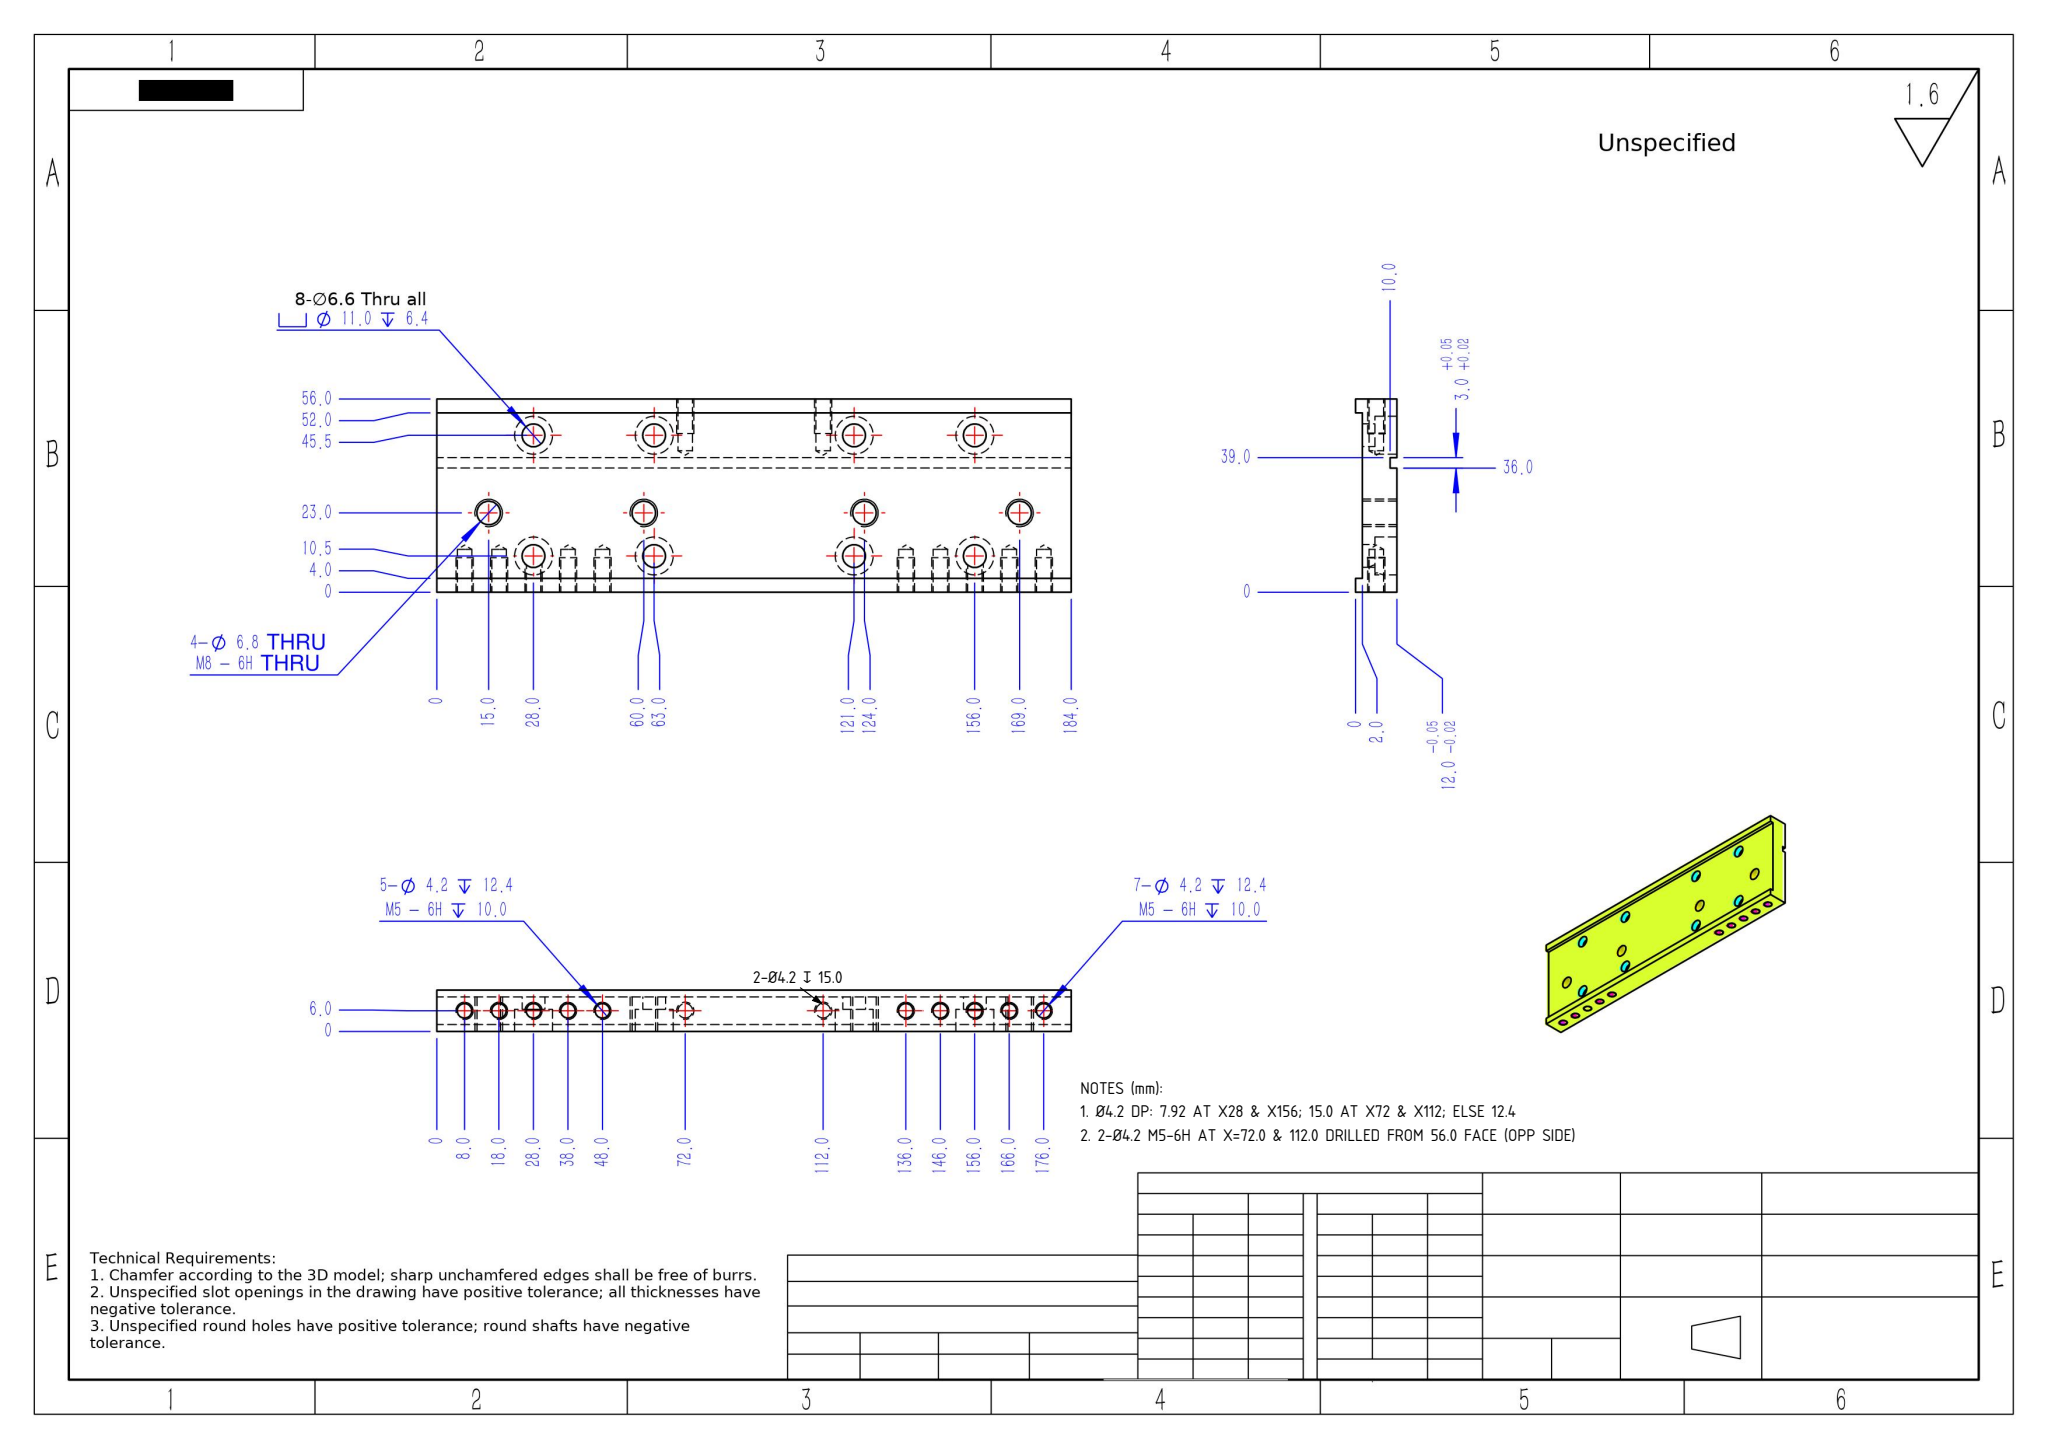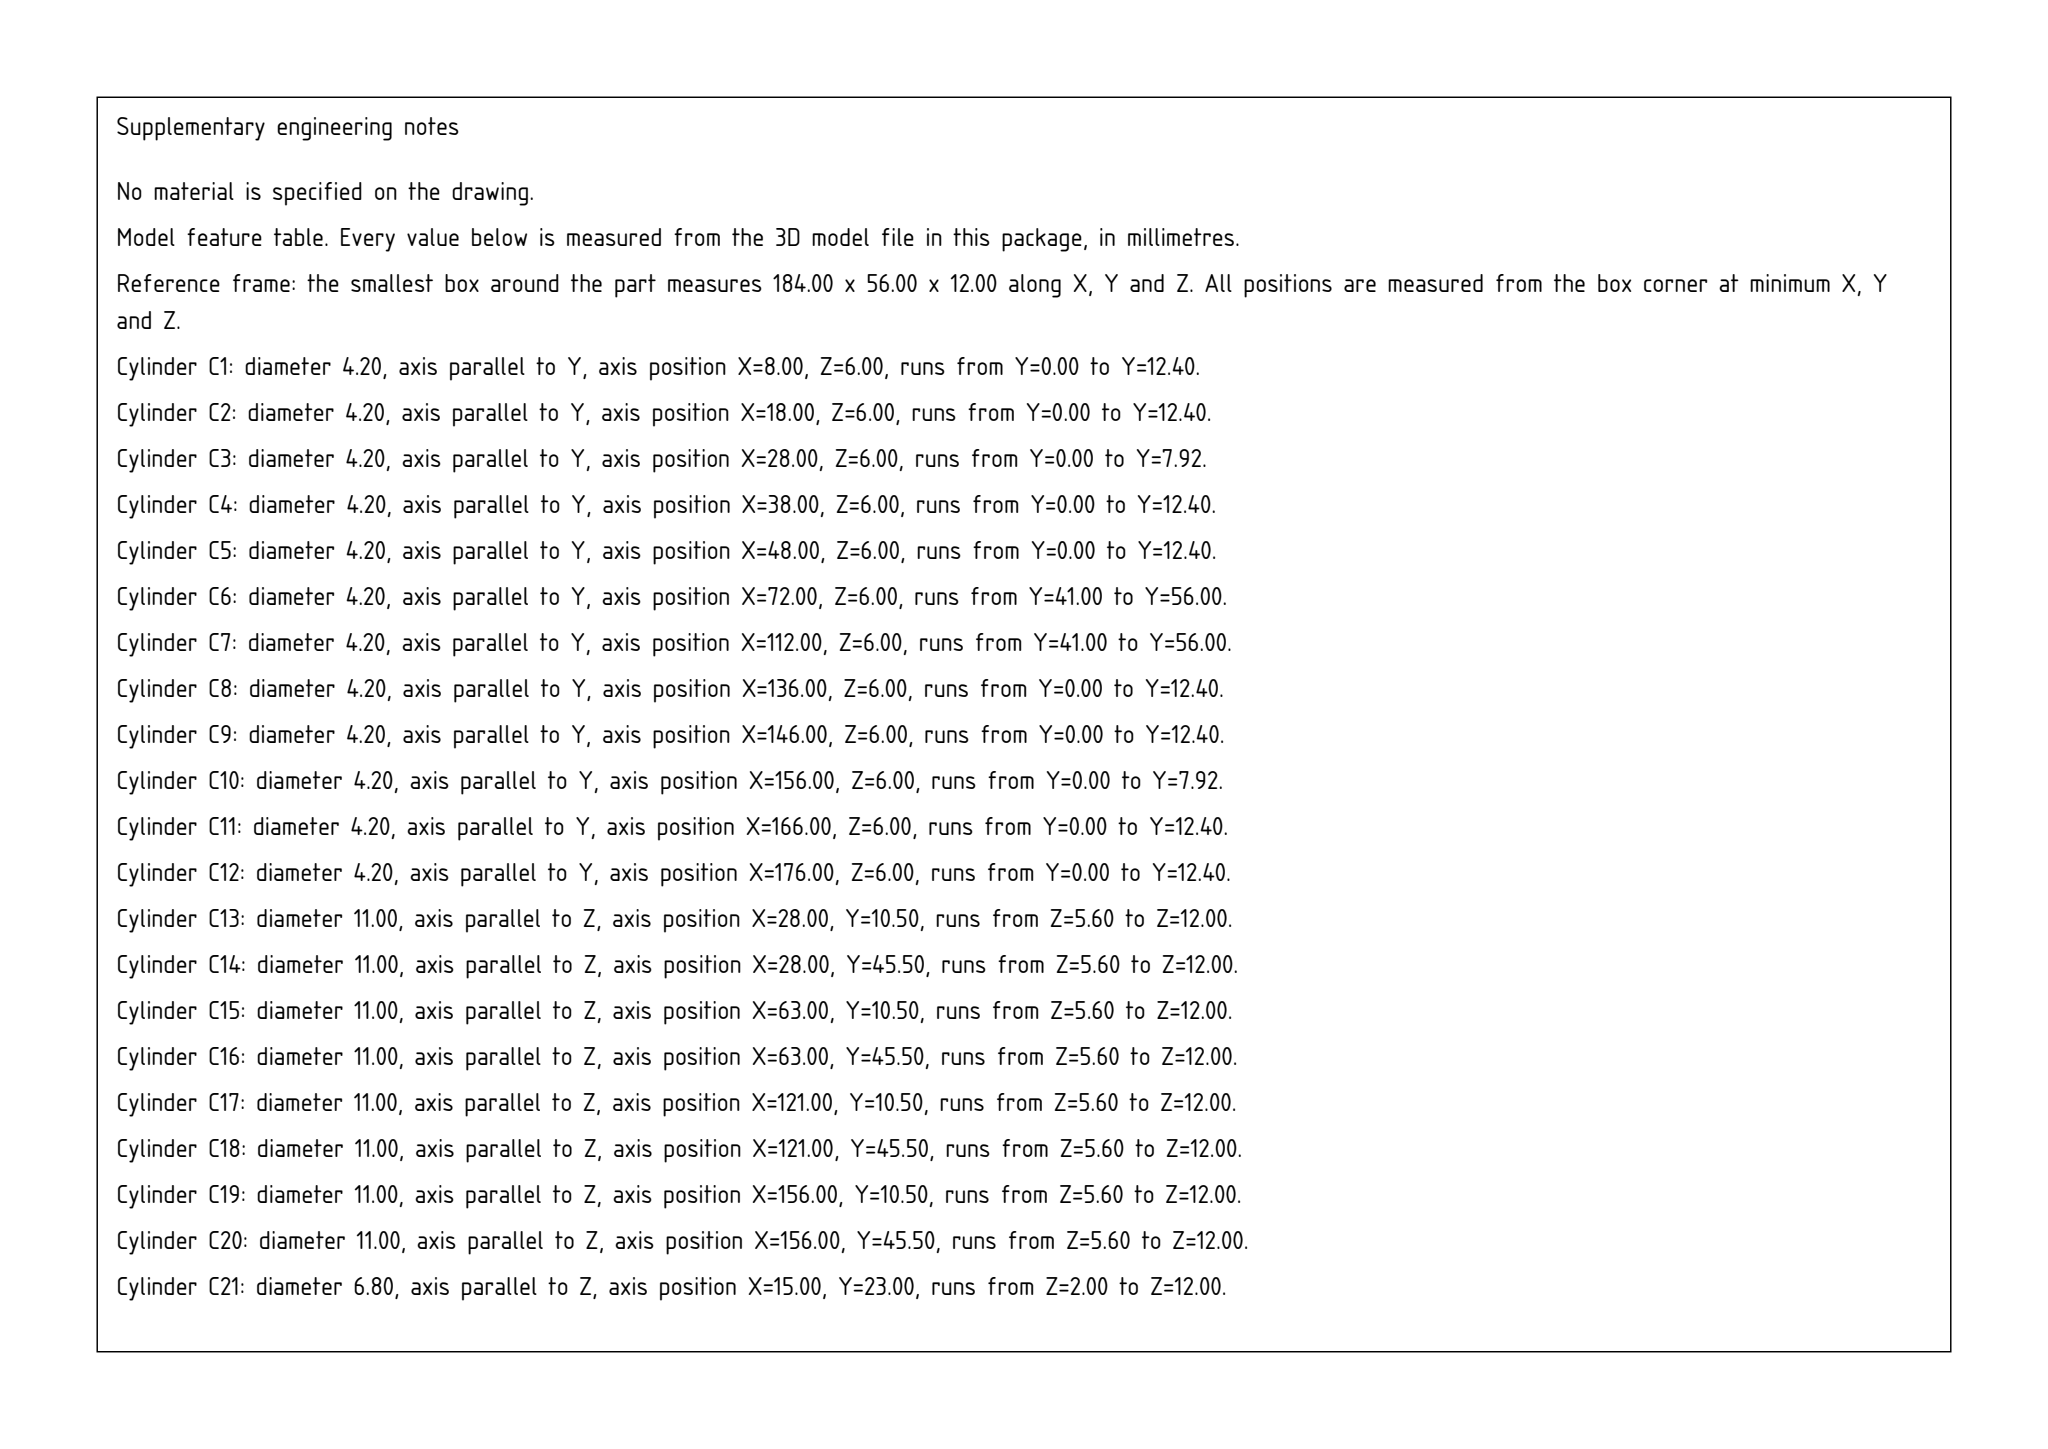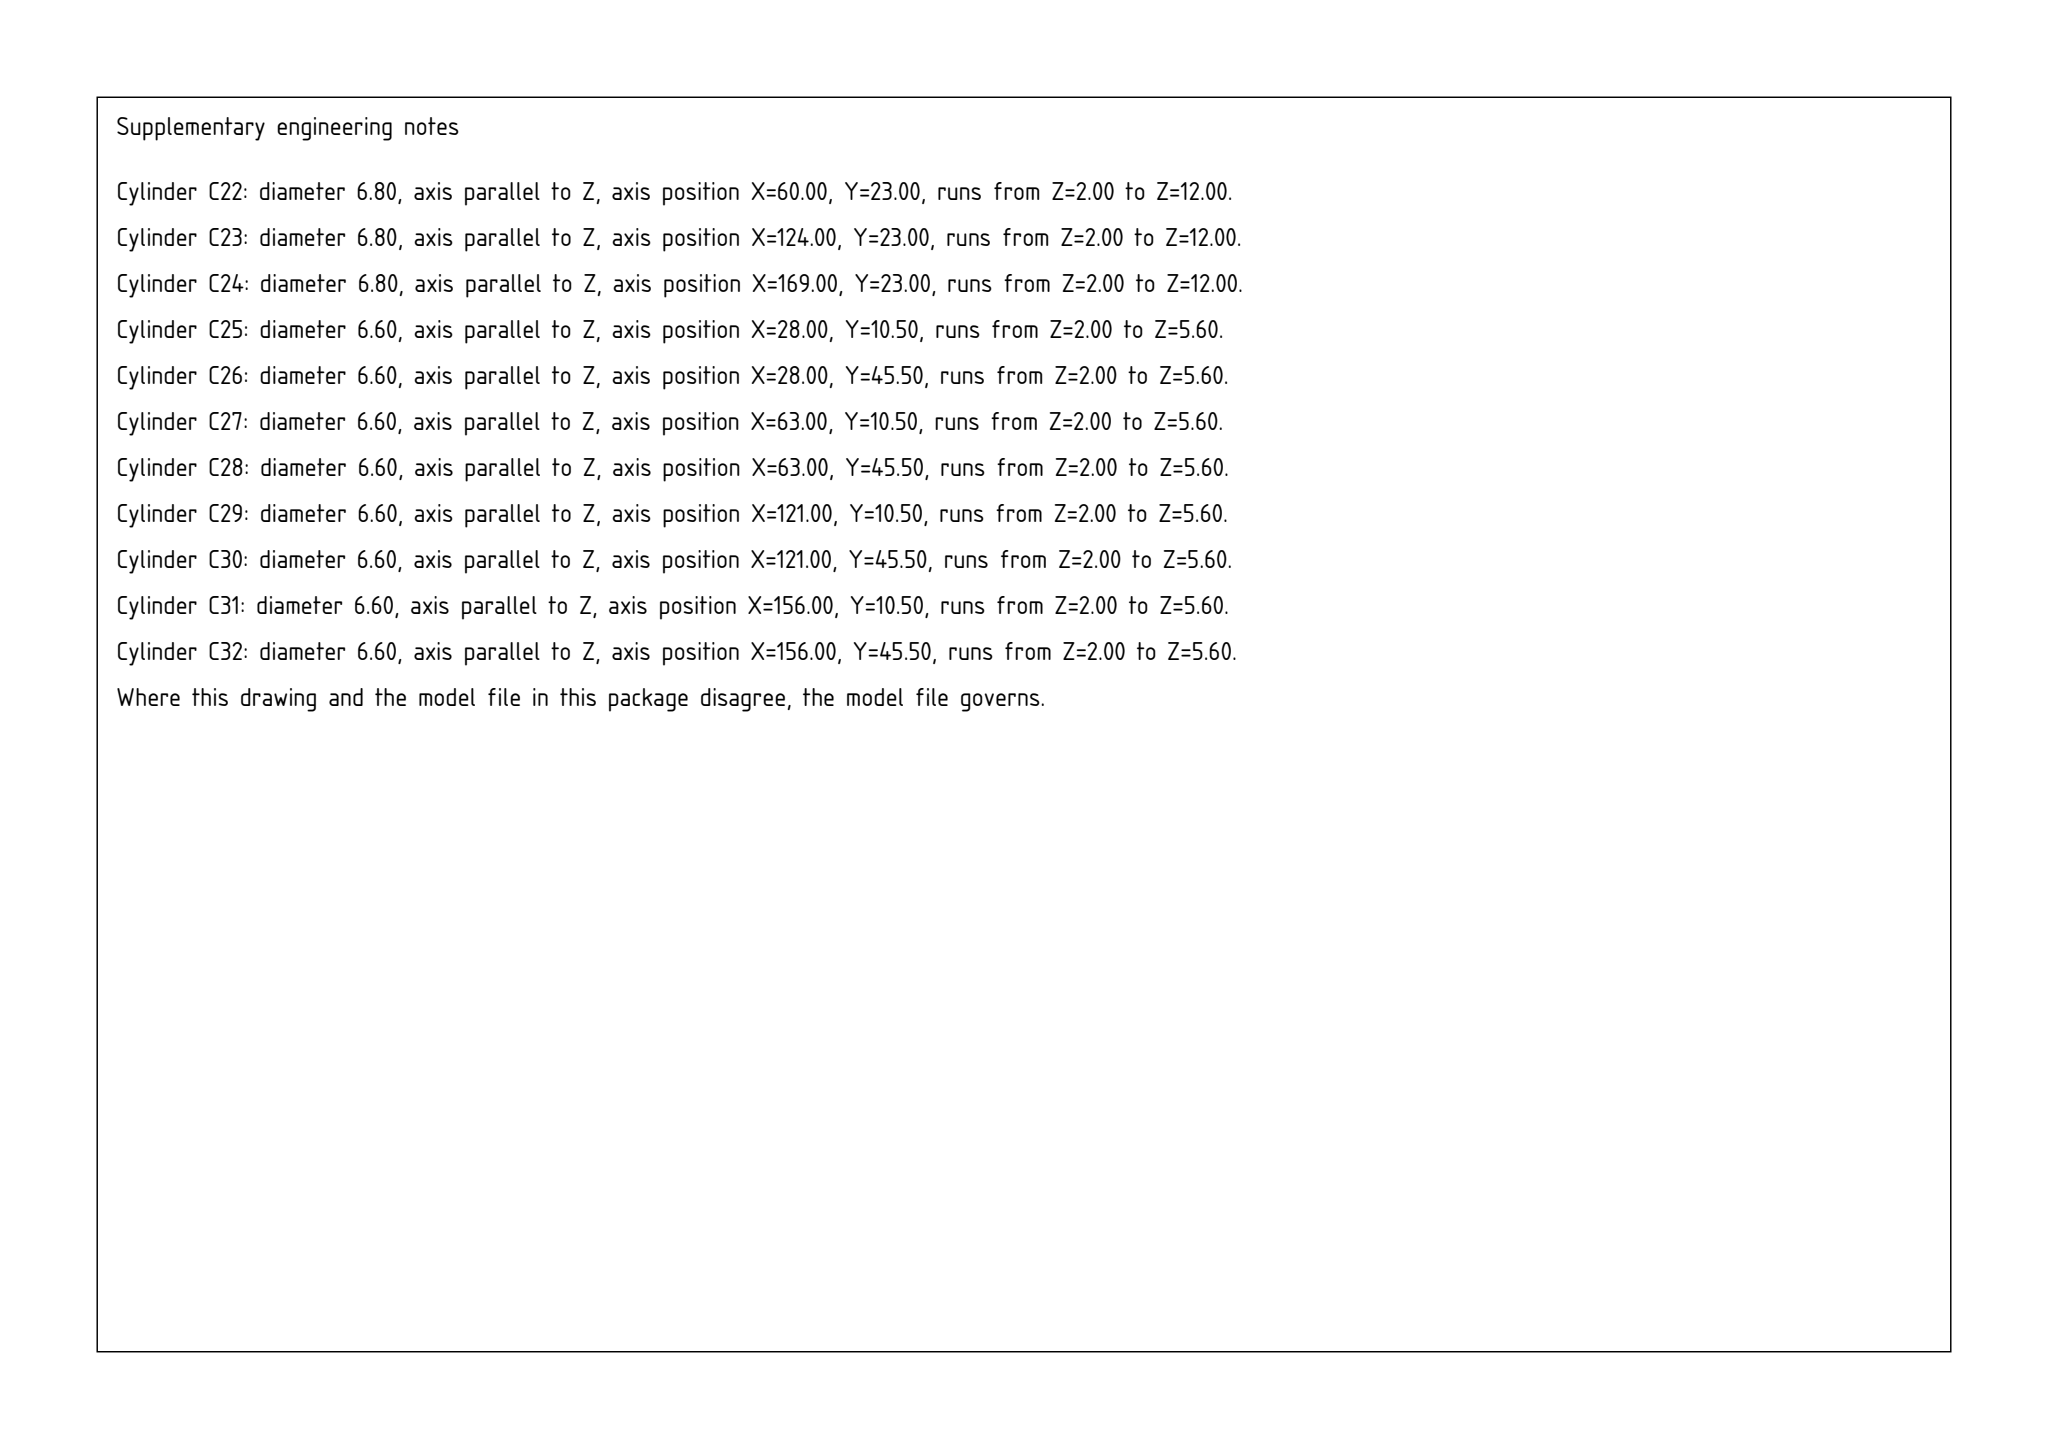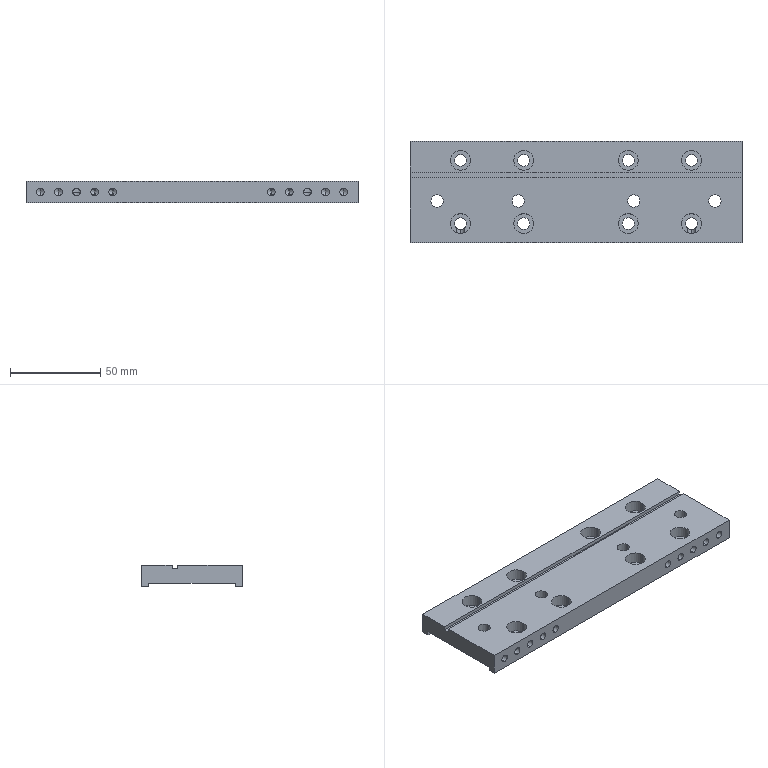Part | SolidWorks | mm | 1 solid | 106 faces | box 184 x 56 x 12 mm | volume 95563 mm3 | cylinder 64 | plane 22 | cone 20 | commonest cylinder face diameters 4.2 x24 11 x16 6.6 x16 6.8 x8
Drawing notes:
Ø4.2 DP: 7.92 AT X28 & X156; 15.0 AT X72 & X112; ELSE 12.4 | from the solid: cyl dia 4.2 lengths: 7.92 at x=28,156; 15.0 at x=72,112; 12.4 at others
2-Ø4.2 M5-6H AT X=72.0 & 112.0 DRILLED FROM 56.0 FACE (OPP SIDE) | from the solid: Ø4.2 holes axis y at x=112.0,z=6.0 and x=72.0,z=6.0 run from y=41.0 to y=56.0; all other ten Ø4.2 holes run y=0.0 to 12.4
2-Ø4.2 AT X=72.0 & 112.0: DP 15.0 (NOT DP 12.4) | from the solid: cylinders dia 4.2 axis y at x=72.0 and x=112.0 from 41.0 to 56.0 = 15.0 full-dia depth
build123d program:
from build123d import *

# Parameters (mm, degrees)
SKETCH1_W                                       = 184
SKETCH1_H                                       = 56
BOSS_EXTRUDE1_DEPTH                             = 6
SKETCH2_W                                       = 184
SKETCH2_H                                       = 48
CUT_EXTRUDE1_DEPTH                              = 2
SKETCH3_W                                       = 184
SKETCH3_H                                       = 3
CUT_EXTRUDE2_DEPTH                              = 2
M6_HEX_SOCKET_HEAD_CAP_SCREW_CBORE1_D           = 6.6
M6_HEX_SOCKET_HEAD_CAP_SCREW_CBORE1_DEPTH       = 12
M6_HEX_SOCKET_HEAD_CAP_SCREW_CBORE1_CBORE_D     = 11
M6_HEX_SOCKET_HEAD_CAP_SCREW_CBORE1_CBORE_DEPTH = 6.4
M8_TAPPED_HOLE1_D                               = 6.8
LPATTERN1_COUNT                                 = 5
LPATTERN1_PITCH                                 = 10
M5_TAPPED_HOLE2_D                               = 4.2
M5_TAPPED_HOLE2_DEPTH                           = 15
M5_TAPPED_HOLE2_TIP                             = 1.262


with BuildPart() as part:
    # Sketch1 → Boss-Extrude1 (new, symmetric)
    with BuildSketch(Plane.XY):
        Rectangle(SKETCH1_W, SKETCH1_H)
    extrude(amount=BOSS_EXTRUDE1_DEPTH, both=True)

    # Sketch2 → Cut-Extrude1 (cut)
    with BuildSketch(Plane(origin=(0, 0, -6), x_dir=(-1, 0, 0), z_dir=(0, 0, -1))):
        Rectangle(SKETCH2_W, SKETCH2_H)
    extrude(amount=-CUT_EXTRUDE1_DEPTH, mode=Mode.SUBTRACT)

    # Sketch3 → Cut-Extrude2 (cut)
    with BuildSketch(Plane.XY.offset(6)):
        with Locations((0, 9.5)):
            Rectangle(SKETCH3_W, SKETCH3_H)
    extrude(amount=-CUT_EXTRUDE2_DEPTH, mode=Mode.SUBTRACT)

    # M6 Hex Socket Head Cap Screw CBORE1
    with Locations(Plane.XY.offset(6)):
        with Locations((-64, 17.5), (-29, 17.5), (-64, -17.5), (-29, -17.5), (29, -17.5), (64, -17.5), (29, 17.5), (64, 17.5)):
            CounterBoreHole(M6_HEX_SOCKET_HEAD_CAP_SCREW_CBORE1_D / 2, M6_HEX_SOCKET_HEAD_CAP_SCREW_CBORE1_CBORE_D / 2, M6_HEX_SOCKET_HEAD_CAP_SCREW_CBORE1_CBORE_DEPTH, depth=M6_HEX_SOCKET_HEAD_CAP_SCREW_CBORE1_DEPTH)

    # M8 Tapped Hole1 (through all)
    with Locations(Plane.XY.offset(6)):
        with Locations((32, -5), (-77, -5), (-32, -5), (77, -5)):
            Hole(M8_TAPPED_HOLE1_D / 2)

    # Sketch9 → M5 Tapped Hole1 (revolve, cut)
    with BuildSketch(Plane(origin=(-84, -28, 0), x_dir=(0, 0, -1), z_dir=(1, 0, 0))):
        Polygon((0, 0), (0, 13.662), (2.1, 12.4), (2.1, 0), align=None)
    m5_tapped_hole1 = revolve(axis=Axis((-84, -34.35, 0), (0, 1, 0)), mode=Mode.SUBTRACT)

    # LPattern1: M5 Tapped Hole1 ×5
    with Locations(*[(i * LPATTERN1_PITCH, 0, 0) for i in range(1, LPATTERN1_COUNT)]):
        add(m5_tapped_hole1, mode=Mode.SUBTRACT)

    # Mirror1: M5 Tapped Hole1 across plane
    add(m5_tapped_hole1.mirror(Plane(origin=(0, 0, 0), x_dir=(0, 0, 1), z_dir=(1, 0, 0))), mode=Mode.SUBTRACT)

    # Mirror1 copy 1 sketch → Mirror1 copy 1 (revolve, cut)
    with BuildSketch(Plane(origin=(74, -28, 0), x_dir=(0, 0, -1), z_dir=(-1, 0, 0))):
        Polygon((0, 0), (0, -13.662), (2.1, -12.4), (2.1, 0), align=None)
    revolve(axis=Axis((74, -34.35, 0), (0, -1, 0)), mode=Mode.SUBTRACT)

    # Mirror1 copy 2 sketch → Mirror1 copy 2 (revolve, cut)
    with BuildSketch(Plane(origin=(64, -28, 0), x_dir=(0, 0, -1), z_dir=(-1, 0, 0))):
        Polygon((0, 0), (0, -13.662), (2.1, -12.4), (2.1, 0), align=None)
    revolve(axis=Axis((64, -34.35, 0), (0, -1, 0)), mode=Mode.SUBTRACT)

    # Mirror1 copy 3 sketch → Mirror1 copy 3 (revolve, cut)
    with BuildSketch(Plane(origin=(54, -28, 0), x_dir=(0, 0, -1), z_dir=(-1, 0, 0))):
        Polygon((0, 0), (0, -13.662), (2.1, -12.4), (2.1, 0), align=None)
    revolve(axis=Axis((54, -34.35, 0), (0, -1, 0)), mode=Mode.SUBTRACT)

    # Mirror1 copy 4 sketch → Mirror1 copy 4 (revolve, cut)
    with BuildSketch(Plane(origin=(44, -28, 0), x_dir=(0, 0, -1), z_dir=(-1, 0, 0))):
        Polygon((0, 0), (0, -13.662), (2.1, -12.4), (2.1, 0), align=None)
    revolve(axis=Axis((44, -34.35, 0), (0, -1, 0)), mode=Mode.SUBTRACT)

    # M5 Tapped Hole2
    with Locations(Plane(origin=(0, 28, 0), x_dir=(1, 0, 0), z_dir=(0, 1, 0))):
        with Locations((20, 0), (-20, 0)):
            Hole(M5_TAPPED_HOLE2_D / 2, depth=M5_TAPPED_HOLE2_DEPTH)
            with Locations((0, 0, -(M5_TAPPED_HOLE2_DEPTH + M5_TAPPED_HOLE2_TIP / 2))):  # 118° drill point
                Cone(0, M5_TAPPED_HOLE2_D / 2, M5_TAPPED_HOLE2_TIP, mode=Mode.SUBTRACT)


solid = part.part